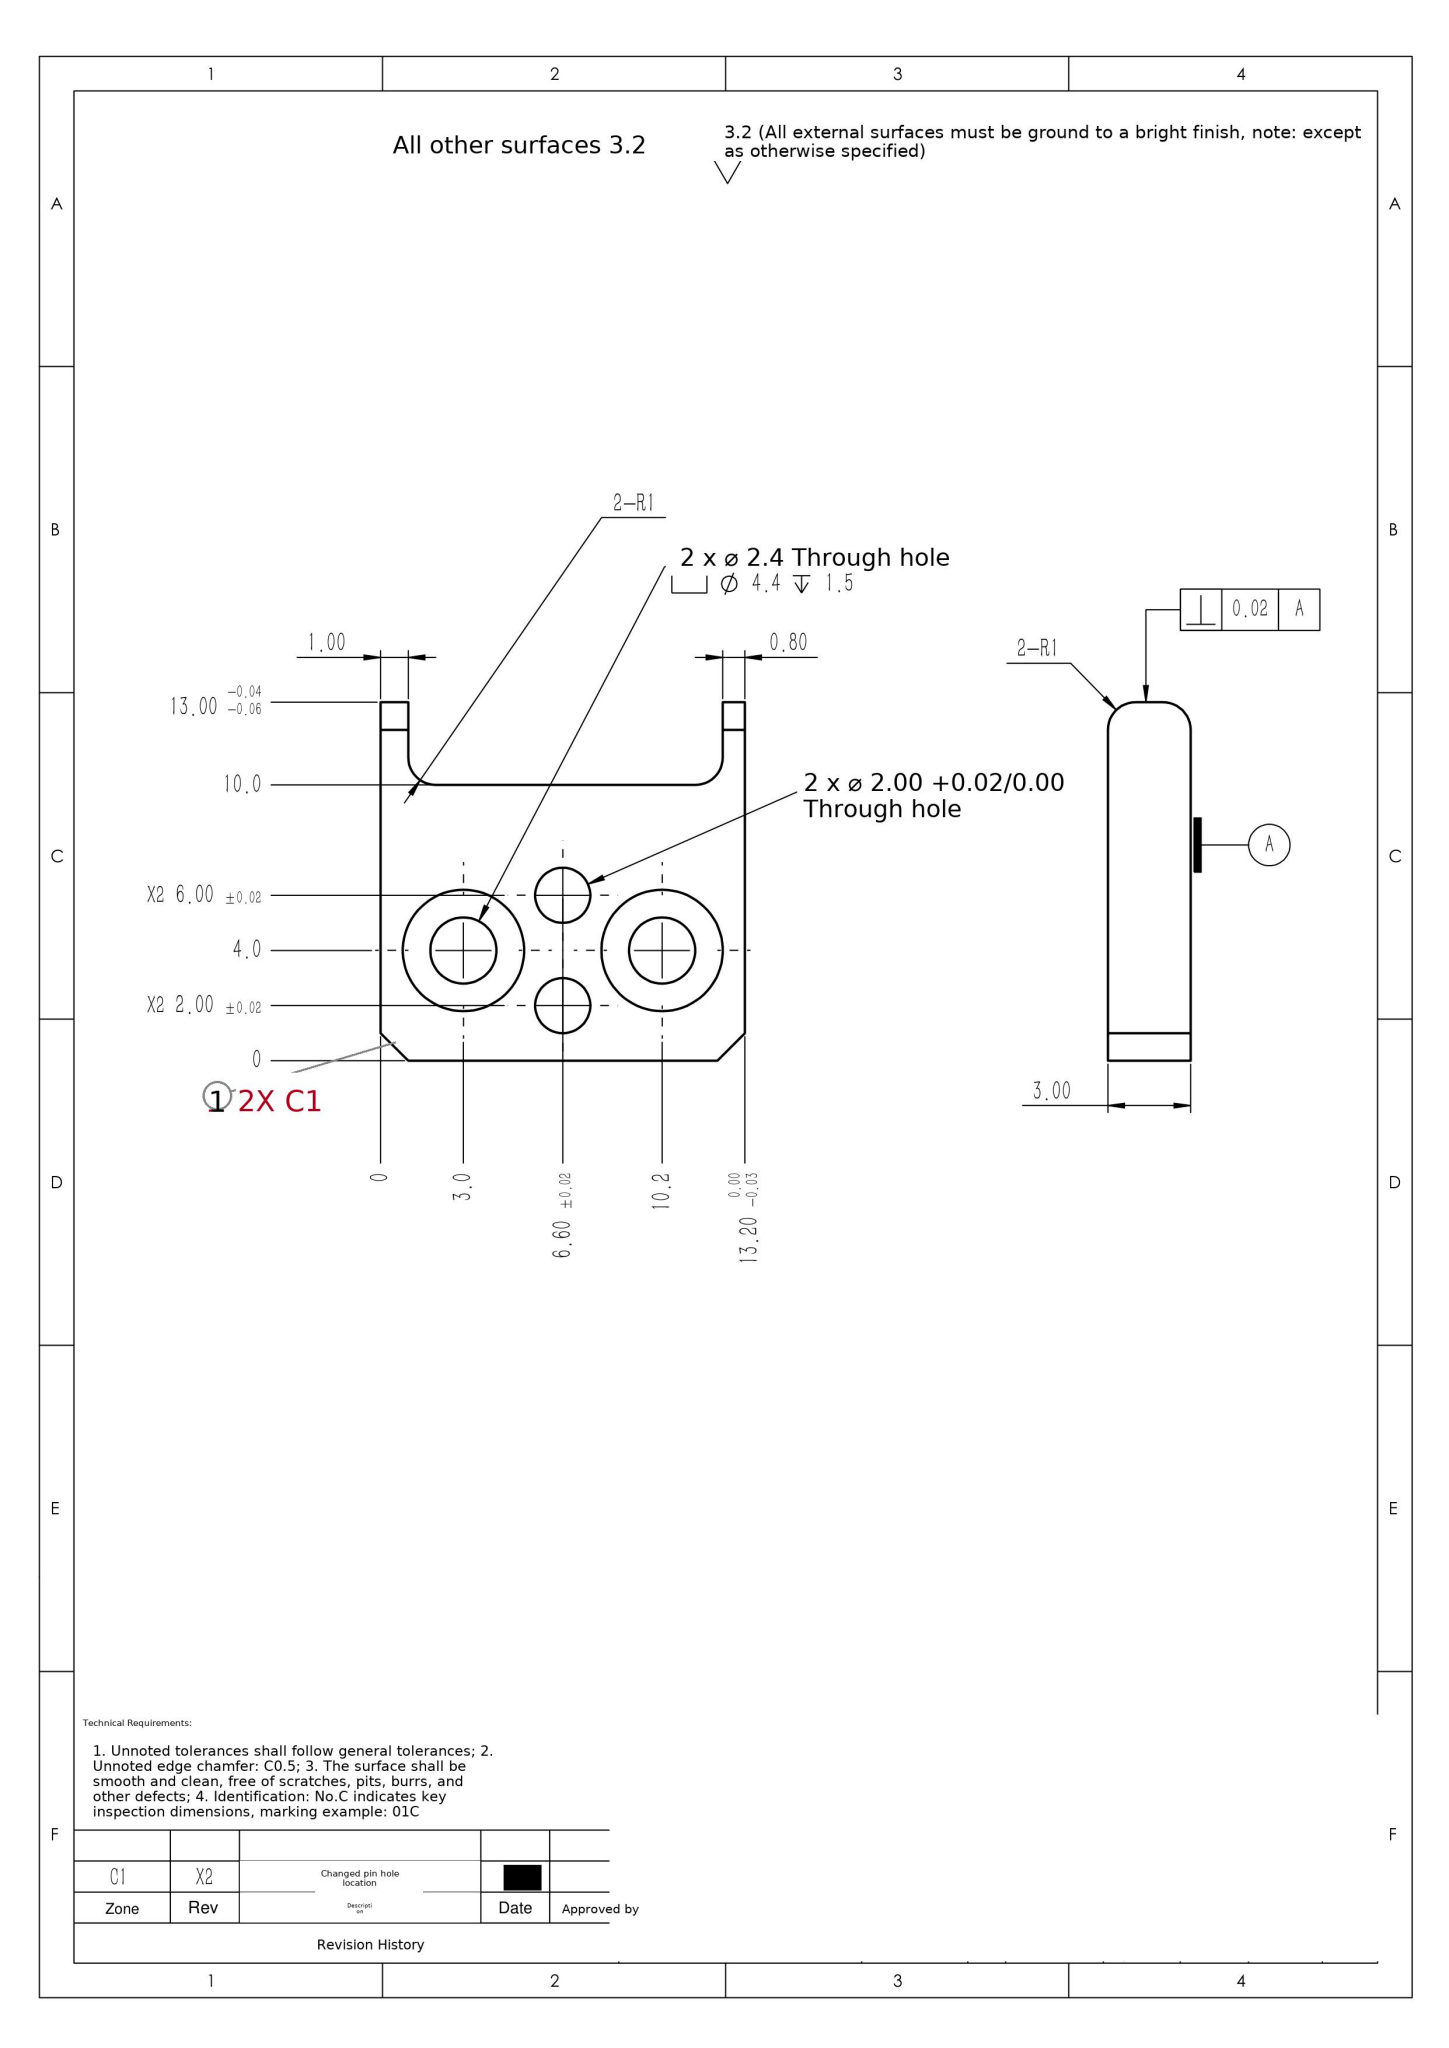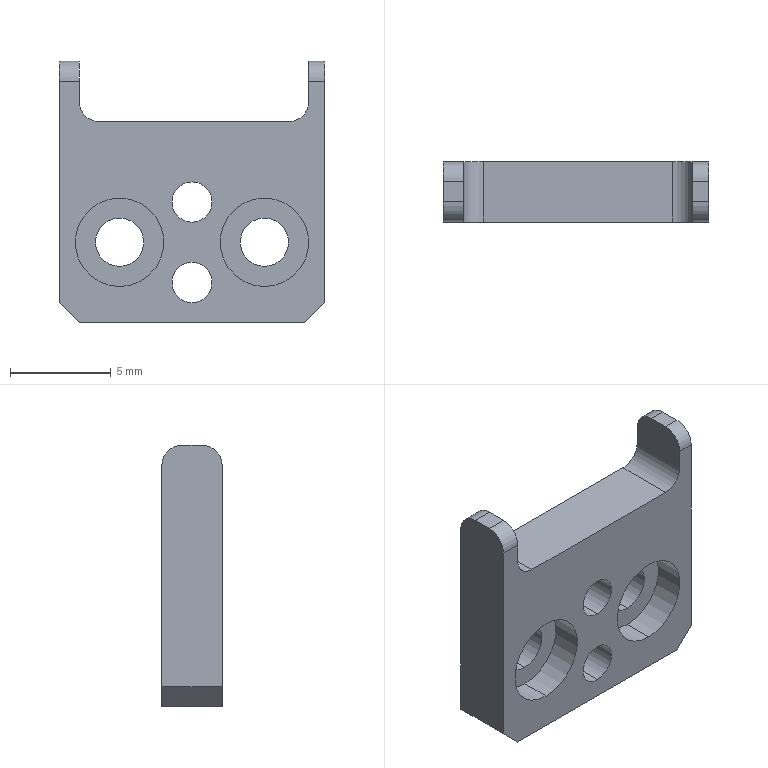Part | SolidWorks | mm | 1 solid | 32 faces | box 13.2 x 3 x 13 mm | volume 332 mm3 | cylinder 18 | plane 14 | commonest cylinder face diameters 2 x10 4.4 x4 2.4 x4
STEP:
#1=CARTESIAN_POINT('',(0.,3.,0.5));
#2=VERTEX_POINT('',#1);
#3=CARTESIAN_POINT('',(0.,3.,-1.5));
#4=VERTEX_POINT('',#3);
#5=CARTESIAN_POINT('',(0.,3.,-0.5));
#6=DIRECTION('',(0.,-1.,0.));
#7=DIRECTION('',(0.,0.,-1.));
#8=AXIS2_PLACEMENT_3D('',#5,#6,#7);
#9=CIRCLE('',#8,1.);
#10=EDGE_CURVE('',#2,#4,#9,.T.);
#11=ORIENTED_EDGE('',*,*,#10,.F.);
#12=CARTESIAN_POINT('',(0.,-0.,0.5));
#13=VERTEX_POINT('',#12);
#14=CARTESIAN_POINT('',(0.,0.,0.5));
#15=DIRECTION('',(0.,-1.,0.));
#16=VECTOR('',#15,1000.);
#17=LINE('',#14,#16);
#18=EDGE_CURVE('',#2,#13,#17,.T.);
#19=ORIENTED_EDGE('',*,*,#18,.T.);
#20=CARTESIAN_POINT('',(0.,-0.,-1.5));
#21=VERTEX_POINT('',#20);
#22=CARTESIAN_POINT('',(0.,-0.,-0.5));
#23=DIRECTION('',(0.,-1.,0.));
#24=DIRECTION('',(0.,0.,-1.));
#25=AXIS2_PLACEMENT_3D('',#22,#23,#24);
#26=CIRCLE('',#25,1.);
#27=EDGE_CURVE('',#13,#21,#26,.T.);
#28=ORIENTED_EDGE('',*,*,#27,.T.);
#29=CARTESIAN_POINT('',(0.,0.,-1.5));
#30=DIRECTION('',(0.,-1.,0.));
#31=VECTOR('',#30,1000.);
#32=LINE('',#29,#31);
#33=EDGE_CURVE('',#4,#21,#32,.T.);
#34=ORIENTED_EDGE('',*,*,#33,.F.);
#35=EDGE_LOOP('',(#11,#19,#28,#34));
#36=FACE_OUTER_BOUND('',#35,.T.);
#37=CARTESIAN_POINT('',(0.,0.,-0.5));
#38=DIRECTION('',(0.,-1.,0.));
#39=DIRECTION('',(0.,0.,-1.));
#40=AXIS2_PLACEMENT_3D('',#37,#38,#39);
#41=CYLINDRICAL_SURFACE('',#40,1.);
#42=ADVANCED_FACE('',(#36),#41,.F.);
#43=CARTESIAN_POINT('',(0.,3.,-3.5));
#44=VERTEX_POINT('',#43);
#45=CARTESIAN_POINT('',(0.,3.,-5.5));
#46=VERTEX_POINT('',#45);
#47=CARTESIAN_POINT('',(0.,3.,-4.5));
#48=DIRECTION('',(0.,-1.,0.));
#49=DIRECTION('',(0.,0.,-1.));
#50=AXIS2_PLACEMENT_3D('',#47,#48,#49);
#51=CIRCLE('',#50,1.);
#52=EDGE_CURVE('',#44,#46,#51,.T.);
#53=ORIENTED_EDGE('',*,*,#52,.F.);
#54=CARTESIAN_POINT('',(0.,-0.,-3.5));
#55=VERTEX_POINT('',#54);
#56=CARTESIAN_POINT('',(0.,0.,-3.5));
#57=DIRECTION('',(0.,-1.,0.));
#58=VECTOR('',#57,1000.);
#59=LINE('',#56,#58);
#60=EDGE_CURVE('',#44,#55,#59,.T.);
#61=ORIENTED_EDGE('',*,*,#60,.T.);
#62=CARTESIAN_POINT('',(0.,-0.,-5.5));
#63=VERTEX_POINT('',#62);
#64=CARTESIAN_POINT('',(0.,-0.,-4.5));
#65=DIRECTION('',(0.,-1.,0.));
#66=DIRECTION('',(0.,0.,-1.));
#67=AXIS2_PLACEMENT_3D('',#64,#65,#66);
#68=CIRCLE('',#67,1.);
#69=EDGE_CURVE('',#55,#63,#68,.T.);
#70=ORIENTED_EDGE('',*,*,#69,.T.);
#71=CARTESIAN_POINT('',(0.,0.,-5.5));
#72=DIRECTION('',(0.,-1.,0.));
#73=VECTOR('',#72,1000.);
#74=LINE('',#71,#73);
#75=EDGE_CURVE('',#46,#63,#74,.T.);
#76=ORIENTED_EDGE('',*,*,#75,.F.);
#77=EDGE_LOOP('',(#53,#61,#70,#76));
#78=FACE_OUTER_BOUND('',#77,.T.);
#79=CARTESIAN_POINT('',(0.,0.,-4.5));
#80=DIRECTION('',(0.,-1.,0.));
#81=DIRECTION('',(0.,0.,-1.));
#82=AXIS2_PLACEMENT_3D('',#79,#80,#81);
#83=CYLINDRICAL_SURFACE('',#82,1.);
#84=ADVANCED_FACE('',(#78),#83,.F.);
#85=CARTESIAN_POINT('',(-3.6,1.5,-0.3));
#86=VERTEX_POINT('',#85);
#87=CARTESIAN_POINT('',(-3.6,1.5,-4.7));
#88=VERTEX_POINT('',#87);
#89=CARTESIAN_POINT('',(-3.6,1.5,-2.5));
#90=DIRECTION('',(0.,-1.,0.));
#91=DIRECTION('',(0.,0.,-1.));
#92=AXIS2_PLACEMENT_3D('',#89,#90,#91);
#93=CIRCLE('',#92,2.2);
#94=EDGE_CURVE('',#86,#88,#93,.T.);
#95=ORIENTED_EDGE('',*,*,#94,.F.);
#96=CARTESIAN_POINT('',(-3.6,0.,-0.3));
#97=VERTEX_POINT('',#96);
#98=CARTESIAN_POINT('',(-3.6,0.,-0.3));
#99=DIRECTION('',(0.,-1.,0.));
#100=VECTOR('',#99,1000.);
#101=LINE('',#98,#100);
#102=EDGE_CURVE('',#86,#97,#101,.T.);
#103=ORIENTED_EDGE('',*,*,#102,.T.);
#104=CARTESIAN_POINT('',(-3.6,0.,-4.7));
#105=VERTEX_POINT('',#104);
#106=CARTESIAN_POINT('',(-3.6,0.,-2.5));
#107=DIRECTION('',(0.,-1.,0.));
#108=DIRECTION('',(0.,0.,-1.));
#109=AXIS2_PLACEMENT_3D('',#106,#107,#108);
#110=CIRCLE('',#109,2.2);
#111=EDGE_CURVE('',#97,#105,#110,.T.);
#112=ORIENTED_EDGE('',*,*,#111,.T.);
#113=CARTESIAN_POINT('',(-3.6,0.,-4.7));
#114=DIRECTION('',(0.,-1.,0.));
#115=VECTOR('',#114,1000.);
#116=LINE('',#113,#115);
#117=EDGE_CURVE('',#88,#105,#116,.T.);
#118=ORIENTED_EDGE('',*,*,#117,.F.);
#119=EDGE_LOOP('',(#95,#103,#112,#118));
#120=FACE_OUTER_BOUND('',#119,.T.);
#121=CARTESIAN_POINT('',(-3.6,0.,-2.5));
#122=DIRECTION('',(0.,-1.,0.));
#123=DIRECTION('',(0.,0.,-1.));
#124=AXIS2_PLACEMENT_3D('',#121,#122,#123);
#125=CYLINDRICAL_SURFACE('',#124,2.2);
#126=ADVANCED_FACE('',(#120),#125,.F.);
#127=CARTESIAN_POINT('',(-3.6,3.,-1.3));
#128=VERTEX_POINT('',#127);
#129=CARTESIAN_POINT('',(-3.6,3.,-3.7));
#130=VERTEX_POINT('',#129);
#131=CARTESIAN_POINT('',(-3.6,3.,-2.5));
#132=DIRECTION('',(0.,-1.,0.));
#133=DIRECTION('',(0.,0.,-1.));
#134=AXIS2_PLACEMENT_3D('',#131,#132,#133);
#135=CIRCLE('',#134,1.2);
#136=EDGE_CURVE('',#128,#130,#135,.T.);
#137=ORIENTED_EDGE('',*,*,#136,.F.);
#138=CARTESIAN_POINT('',(-3.6,1.5,-1.3));
#139=VERTEX_POINT('',#138);
#140=CARTESIAN_POINT('',(-3.6,0.,-1.3));
#141=DIRECTION('',(0.,-1.,0.));
#142=VECTOR('',#141,1000.);
#143=LINE('',#140,#142);
#144=EDGE_CURVE('',#128,#139,#143,.T.);
#145=ORIENTED_EDGE('',*,*,#144,.T.);
#146=CARTESIAN_POINT('',(-3.6,1.5,-3.7));
#147=VERTEX_POINT('',#146);
#148=CARTESIAN_POINT('',(-3.6,1.5,-2.5));
#149=DIRECTION('',(0.,-1.,0.));
#150=DIRECTION('',(0.,0.,-1.));
#151=AXIS2_PLACEMENT_3D('',#148,#149,#150);
#152=CIRCLE('',#151,1.2);
#153=EDGE_CURVE('',#139,#147,#152,.T.);
#154=ORIENTED_EDGE('',*,*,#153,.T.);
#155=CARTESIAN_POINT('',(-3.6,0.,-3.7));
#156=DIRECTION('',(0.,-1.,0.));
#157=VECTOR('',#156,1000.);
#158=LINE('',#155,#157);
#159=EDGE_CURVE('',#130,#147,#158,.T.);
#160=ORIENTED_EDGE('',*,*,#159,.F.);
#161=EDGE_LOOP('',(#137,#145,#154,#160));
#162=FACE_OUTER_BOUND('',#161,.T.);
#163=CARTESIAN_POINT('',(-3.6,0.,-2.5));
#164=DIRECTION('',(0.,-1.,0.));
#165=DIRECTION('',(0.,0.,-1.));
#166=AXIS2_PLACEMENT_3D('',#163,#164,#165);
#167=CYLINDRICAL_SURFACE('',#166,1.2);
#168=ADVANCED_FACE('',(#162),#167,.F.);
#169=CARTESIAN_POINT('',(3.6,1.5,-0.3));
#170=VERTEX_POINT('',#169);
#171=CARTESIAN_POINT('',(3.6,1.5,-4.7));
#172=VERTEX_POINT('',#171);
#173=CARTESIAN_POINT('',(3.6,1.5,-2.5));
#174=DIRECTION('',(0.,-1.,0.));
#175=DIRECTION('',(0.,0.,-1.));
#176=AXIS2_PLACEMENT_3D('',#173,#174,#175);
#177=CIRCLE('',#176,2.2);
#178=EDGE_CURVE('',#170,#172,#177,.T.);
#179=ORIENTED_EDGE('',*,*,#178,.F.);
#180=CARTESIAN_POINT('',(3.6,0.,-0.3));
#181=VERTEX_POINT('',#180);
#182=CARTESIAN_POINT('',(3.6,0.,-0.3));
#183=DIRECTION('',(0.,-1.,0.));
#184=VECTOR('',#183,1000.);
#185=LINE('',#182,#184);
#186=EDGE_CURVE('',#170,#181,#185,.T.);
#187=ORIENTED_EDGE('',*,*,#186,.T.);
#188=CARTESIAN_POINT('',(3.6,0.,-4.7));
#189=VERTEX_POINT('',#188);
#190=CARTESIAN_POINT('',(3.6,0.,-2.5));
#191=DIRECTION('',(0.,-1.,0.));
#192=DIRECTION('',(0.,0.,-1.));
#193=AXIS2_PLACEMENT_3D('',#190,#191,#192);
#194=CIRCLE('',#193,2.2);
#195=EDGE_CURVE('',#181,#189,#194,.T.);
#196=ORIENTED_EDGE('',*,*,#195,.T.);
#197=CARTESIAN_POINT('',(3.6,0.,-4.7));
#198=DIRECTION('',(0.,-1.,0.));
#199=VECTOR('',#198,1000.);
#200=LINE('',#197,#199);
#201=EDGE_CURVE('',#172,#189,#200,.T.);
#202=ORIENTED_EDGE('',*,*,#201,.F.);
#203=EDGE_LOOP('',(#179,#187,#196,#202));
#204=FACE_OUTER_BOUND('',#203,.T.);
#205=CARTESIAN_POINT('',(3.6,0.,-2.5));
#206=DIRECTION('',(0.,-1.,0.));
#207=DIRECTION('',(0.,0.,-1.));
#208=AXIS2_PLACEMENT_3D('',#205,#206,#207);
#209=CYLINDRICAL_SURFACE('',#208,2.2);
#210=ADVANCED_FACE('',(#204),#209,.F.);
#211=CARTESIAN_POINT('',(3.6,3.,-1.3));
#212=VERTEX_POINT('',#211);
#213=CARTESIAN_POINT('',(3.6,3.,-3.7));
#214=VERTEX_POINT('',#213);
#215=CARTESIAN_POINT('',(3.6,3.,-2.5));
#216=DIRECTION('',(0.,-1.,0.));
#217=DIRECTION('',(0.,0.,-1.));
#218=AXIS2_PLACEMENT_3D('',#215,#216,#217);
#219=CIRCLE('',#218,1.2);
#220=EDGE_CURVE('',#212,#214,#219,.T.);
#221=ORIENTED_EDGE('',*,*,#220,.F.);
#222=CARTESIAN_POINT('',(3.6,1.5,-1.3));
#223=VERTEX_POINT('',#222);
#224=CARTESIAN_POINT('',(3.6,0.,-1.3));
#225=DIRECTION('',(0.,-1.,0.));
#226=VECTOR('',#225,1000.);
#227=LINE('',#224,#226);
#228=EDGE_CURVE('',#212,#223,#227,.T.);
#229=ORIENTED_EDGE('',*,*,#228,.T.);
#230=CARTESIAN_POINT('',(3.6,1.5,-3.7));
#231=VERTEX_POINT('',#230);
#232=CARTESIAN_POINT('',(3.6,1.5,-2.5));
#233=DIRECTION('',(0.,-1.,0.));
#234=DIRECTION('',(0.,0.,-1.));
#235=AXIS2_PLACEMENT_3D('',#232,#233,#234);
#236=CIRCLE('',#235,1.2);
#237=EDGE_CURVE('',#223,#231,#236,.T.);
#238=ORIENTED_EDGE('',*,*,#237,.T.);
#239=CARTESIAN_POINT('',(3.6,0.,-3.7));
#240=DIRECTION('',(0.,-1.,0.));
#241=VECTOR('',#240,1000.);
#242=LINE('',#239,#241);
#243=EDGE_CURVE('',#214,#231,#242,.T.);
#244=ORIENTED_EDGE('',*,*,#243,.F.);
#245=EDGE_LOOP('',(#221,#229,#238,#244));
#246=FACE_OUTER_BOUND('',#245,.T.);
#247=CARTESIAN_POINT('',(3.6,0.,-2.5));
#248=DIRECTION('',(0.,-1.,0.));
#249=DIRECTION('',(0.,0.,-1.));
#250=AXIS2_PLACEMENT_3D('',#247,#248,#249);
#251=CYLINDRICAL_SURFACE('',#250,1.2);
#252=ADVANCED_FACE('',(#246),#251,.F.);
#253=CARTESIAN_POINT('',(0.,3.,-0.5));
#254=DIRECTION('',(0.,-1.,0.));
#255=DIRECTION('',(0.,0.,-1.));
#256=AXIS2_PLACEMENT_3D('',#253,#254,#255);
#257=CIRCLE('',#256,1.);
#258=EDGE_CURVE('',#4,#2,#257,.T.);
#259=ORIENTED_EDGE('',*,*,#258,.T.);
#260=ORIENTED_EDGE('',*,*,#10,.T.);
#261=EDGE_LOOP('',(#259,#260));
#262=FACE_BOUND('',#261,.T.);
#263=CARTESIAN_POINT('',(0.,3.,-4.5));
#264=DIRECTION('',(0.,-1.,0.));
#265=DIRECTION('',(0.,0.,-1.));
#266=AXIS2_PLACEMENT_3D('',#263,#264,#265);
#267=CIRCLE('',#266,1.);
#268=EDGE_CURVE('',#46,#44,#267,.T.);
#269=ORIENTED_EDGE('',*,*,#268,.T.);
#270=ORIENTED_EDGE('',*,*,#52,.T.);
#271=EDGE_LOOP('',(#269,#270));
#272=FACE_BOUND('',#271,.T.);
#273=CARTESIAN_POINT('',(6.6,3.,5.5));
#274=VERTEX_POINT('',#273);
#275=CARTESIAN_POINT('',(6.6,3.,-5.5));
#276=VERTEX_POINT('',#275);
#277=CARTESIAN_POINT('',(6.6,3.,-6.5));
#278=DIRECTION('',(-0.,0.,-1.));
#279=VECTOR('',#278,1000.);
#280=LINE('',#277,#279);
#281=EDGE_CURVE('',#274,#276,#280,.T.);
#282=ORIENTED_EDGE('',*,*,#281,.T.);
#283=CARTESIAN_POINT('',(5.6,3.,-6.5));
#284=VERTEX_POINT('',#283);
#285=CARTESIAN_POINT('',(6.05,3.,-6.05));
#286=DIRECTION('',(-0.7071,0.,-0.7071));
#287=VECTOR('',#286,1000.);
#288=LINE('',#285,#287);
#289=EDGE_CURVE('',#276,#284,#288,.T.);
#290=ORIENTED_EDGE('',*,*,#289,.T.);
#291=CARTESIAN_POINT('',(-5.6,3.,-6.5));
#292=VERTEX_POINT('',#291);
#293=CARTESIAN_POINT('',(-6.6,3.,-6.5));
#294=DIRECTION('',(-1.,0.,0.));
#295=VECTOR('',#294,1000.);
#296=LINE('',#293,#295);
#297=EDGE_CURVE('',#284,#292,#296,.T.);
#298=ORIENTED_EDGE('',*,*,#297,.T.);
#299=CARTESIAN_POINT('',(-6.6,3.,-5.5));
#300=VERTEX_POINT('',#299);
#301=CARTESIAN_POINT('',(-6.05,3.,-6.05));
#302=DIRECTION('',(-0.7071,0.,0.7071));
#303=VECTOR('',#302,1000.);
#304=LINE('',#301,#303);
#305=EDGE_CURVE('',#292,#300,#304,.T.);
#306=ORIENTED_EDGE('',*,*,#305,.T.);
#307=CARTESIAN_POINT('',(-6.6,3.,5.5));
#308=VERTEX_POINT('',#307);
#309=CARTESIAN_POINT('',(-6.6,3.,-6.5));
#310=DIRECTION('',(0.,0.,1.));
#311=VECTOR('',#310,1000.);
#312=LINE('',#309,#311);
#313=EDGE_CURVE('',#300,#308,#312,.T.);
#314=ORIENTED_EDGE('',*,*,#313,.T.);
#315=CARTESIAN_POINT('',(-5.6,3.,5.5));
#316=VERTEX_POINT('',#315);
#317=CARTESIAN_POINT('',(-5.6,3.,5.5));
#318=DIRECTION('',(1.,0.,0.));
#319=VECTOR('',#318,1000.);
#320=LINE('',#317,#319);
#321=EDGE_CURVE('',#308,#316,#320,.T.);
#322=ORIENTED_EDGE('',*,*,#321,.T.);
#323=CARTESIAN_POINT('',(-5.6,3.,4.5));
#324=VERTEX_POINT('',#323);
#325=CARTESIAN_POINT('',(-5.6,3.,6.5));
#326=DIRECTION('',(0.,0.,-1.));
#327=VECTOR('',#326,1000.);
#328=LINE('',#325,#327);
#329=EDGE_CURVE('',#316,#324,#328,.T.);
#330=ORIENTED_EDGE('',*,*,#329,.T.);
#331=CARTESIAN_POINT('',(-4.6,3.,3.5));
#332=VERTEX_POINT('',#331);
#333=CARTESIAN_POINT('',(-4.6,3.,4.5));
#334=DIRECTION('',(0.,-1.,0.));
#335=DIRECTION('',(0.,0.,1.));
#336=AXIS2_PLACEMENT_3D('',#333,#334,#335);
#337=CIRCLE('',#336,1.);
#338=EDGE_CURVE('',#324,#332,#337,.T.);
#339=ORIENTED_EDGE('',*,*,#338,.T.);
#340=CARTESIAN_POINT('',(4.8,3.,3.5));
#341=VERTEX_POINT('',#340);
#342=CARTESIAN_POINT('',(5.8,3.,3.5));
#343=DIRECTION('',(1.,0.,0.));
#344=VECTOR('',#343,1000.);
#345=LINE('',#342,#344);
#346=EDGE_CURVE('',#332,#341,#345,.T.);
#347=ORIENTED_EDGE('',*,*,#346,.T.);
#348=CARTESIAN_POINT('',(5.8,3.,4.5));
#349=VERTEX_POINT('',#348);
#350=CARTESIAN_POINT('',(4.8,3.,4.5));
#351=DIRECTION('',(0.,-1.,0.));
#352=DIRECTION('',(0.,0.,1.));
#353=AXIS2_PLACEMENT_3D('',#350,#351,#352);
#354=CIRCLE('',#353,1.);
#355=EDGE_CURVE('',#341,#349,#354,.T.);
#356=ORIENTED_EDGE('',*,*,#355,.T.);
#357=CARTESIAN_POINT('',(5.8,3.,5.5));
#358=VERTEX_POINT('',#357);
#359=CARTESIAN_POINT('',(5.8,3.,6.5));
#360=DIRECTION('',(0.,0.,1.));
#361=VECTOR('',#360,1000.);
#362=LINE('',#359,#361);
#363=EDGE_CURVE('',#349,#358,#362,.T.);
#364=ORIENTED_EDGE('',*,*,#363,.T.);
#365=CARTESIAN_POINT('',(6.6,3.,5.5));
#366=DIRECTION('',(1.,0.,0.));
#367=VECTOR('',#366,1000.);
#368=LINE('',#365,#367);
#369=EDGE_CURVE('',#358,#274,#368,.T.);
#370=ORIENTED_EDGE('',*,*,#369,.T.);
#371=EDGE_LOOP('',(#282,#290,#298,#306,#314,#322,#330,#339,#347,#356,#364,#370));
#372=FACE_OUTER_BOUND('',#371,.T.);
#373=CARTESIAN_POINT('',(3.6,3.,-2.5));
#374=DIRECTION('',(0.,-1.,0.));
#375=DIRECTION('',(0.,0.,-1.));
#376=AXIS2_PLACEMENT_3D('',#373,#374,#375);
#377=CIRCLE('',#376,1.2);
#378=EDGE_CURVE('',#214,#212,#377,.T.);
#379=ORIENTED_EDGE('',*,*,#378,.T.);
#380=ORIENTED_EDGE('',*,*,#220,.T.);
#381=EDGE_LOOP('',(#379,#380));
#382=FACE_BOUND('',#381,.T.);
#383=CARTESIAN_POINT('',(-3.6,3.,-2.5));
#384=DIRECTION('',(0.,-1.,0.));
#385=DIRECTION('',(0.,0.,-1.));
#386=AXIS2_PLACEMENT_3D('',#383,#384,#385);
#387=CIRCLE('',#386,1.2);
#388=EDGE_CURVE('',#130,#128,#387,.T.);
#389=ORIENTED_EDGE('',*,*,#388,.T.);
#390=ORIENTED_EDGE('',*,*,#136,.T.);
#391=EDGE_LOOP('',(#389,#390));
#392=FACE_BOUND('',#391,.T.);
#393=CARTESIAN_POINT('',(0.,3.,0.));
#394=DIRECTION('',(0.,1.,0.));
#395=DIRECTION('',(0.,0.,1.));
#396=AXIS2_PLACEMENT_3D('',#393,#394,#395);
#397=PLANE('',#396);
#398=ADVANCED_FACE('',(#262,#272,#372,#382,#392),#397,.T.);
#399=CARTESIAN_POINT('',(6.6,2.,6.5));
#400=VERTEX_POINT('',#399);
#401=CARTESIAN_POINT('',(6.6,1.,6.5));
#402=VERTEX_POINT('',#401);
#403=CARTESIAN_POINT('',(6.6,3.,6.5));
#404=DIRECTION('',(0.,-1.,0.));
#405=VECTOR('',#404,1000.);
#406=LINE('',#403,#405);
#407=EDGE_CURVE('',#400,#402,#406,.T.);
#408=ORIENTED_EDGE('',*,*,#407,.F.);
#409=CARTESIAN_POINT('',(5.8,2.,6.5));
#410=VERTEX_POINT('',#409);
#411=CARTESIAN_POINT('',(5.8,2.,6.5));
#412=DIRECTION('',(-1.,0.,0.));
#413=VECTOR('',#412,1000.);
#414=LINE('',#411,#413);
#415=EDGE_CURVE('',#400,#410,#414,.T.);
#416=ORIENTED_EDGE('',*,*,#415,.T.);
#417=CARTESIAN_POINT('',(5.8,1.,6.5));
#418=VERTEX_POINT('',#417);
#419=CARTESIAN_POINT('',(5.8,3.,6.5));
#420=DIRECTION('',(0.,-1.,0.));
#421=VECTOR('',#420,1000.);
#422=LINE('',#419,#421);
#423=EDGE_CURVE('',#410,#418,#422,.T.);
#424=ORIENTED_EDGE('',*,*,#423,.T.);
#425=CARTESIAN_POINT('',(-6.6,1.,6.5));
#426=DIRECTION('',(1.,0.,0.));
#427=VECTOR('',#426,1000.);
#428=LINE('',#425,#427);
#429=EDGE_CURVE('',#418,#402,#428,.T.);
#430=ORIENTED_EDGE('',*,*,#429,.T.);
#431=EDGE_LOOP('',(#408,#416,#424,#430));
#432=FACE_OUTER_BOUND('',#431,.T.);
#433=CARTESIAN_POINT('',(-6.6,3.,6.5));
#434=DIRECTION('',(0.,0.,-1.));
#435=DIRECTION('',(-1.,0.,0.));
#436=AXIS2_PLACEMENT_3D('',#433,#434,#435);
#437=PLANE('',#436);
#438=ADVANCED_FACE('',(#432),#437,.F.);
#439=CARTESIAN_POINT('',(6.6,0.,5.5));
#440=VERTEX_POINT('',#439);
#441=CARTESIAN_POINT('',(6.6,0.,-5.5));
#442=VERTEX_POINT('',#441);
#443=CARTESIAN_POINT('',(6.6,0.,-6.5));
#444=DIRECTION('',(-0.,0.,-1.));
#445=VECTOR('',#444,1000.);
#446=LINE('',#443,#445);
#447=EDGE_CURVE('',#440,#442,#446,.T.);
#448=ORIENTED_EDGE('',*,*,#447,.T.);
#449=CARTESIAN_POINT('',(6.6,3.,-5.5));
#450=DIRECTION('',(0.,1.,0.));
#451=VECTOR('',#450,1000.);
#452=LINE('',#449,#451);
#453=EDGE_CURVE('',#442,#276,#452,.T.);
#454=ORIENTED_EDGE('',*,*,#453,.T.);
#455=ORIENTED_EDGE('',*,*,#281,.F.);
#456=CARTESIAN_POINT('',(6.6,2.,5.5));
#457=DIRECTION('',(1.,0.,-0.));
#458=DIRECTION('',(0.,0.,1.));
#459=AXIS2_PLACEMENT_3D('',#456,#457,#458);
#460=CIRCLE('',#459,1.);
#461=EDGE_CURVE('',#274,#400,#460,.T.);
#462=ORIENTED_EDGE('',*,*,#461,.T.);
#463=ORIENTED_EDGE('',*,*,#407,.T.);
#464=CARTESIAN_POINT('',(6.6,1.,5.5));
#465=DIRECTION('',(1.,0.,-0.));
#466=DIRECTION('',(0.,0.,1.));
#467=AXIS2_PLACEMENT_3D('',#464,#465,#466);
#468=CIRCLE('',#467,1.);
#469=EDGE_CURVE('',#402,#440,#468,.T.);
#470=ORIENTED_EDGE('',*,*,#469,.T.);
#471=EDGE_LOOP('',(#448,#454,#455,#462,#463,#470));
#472=FACE_OUTER_BOUND('',#471,.T.);
#473=CARTESIAN_POINT('',(6.6,3.,-6.5));
#474=DIRECTION('',(-1.,0.,0.));
#475=DIRECTION('',(0.,0.,1.));
#476=AXIS2_PLACEMENT_3D('',#473,#474,#475);
#477=PLANE('',#476);
#478=ADVANCED_FACE('',(#472),#477,.F.);
#479=ORIENTED_EDGE('',*,*,#297,.F.);
#480=CARTESIAN_POINT('',(5.6,0.,-6.5));
#481=VERTEX_POINT('',#480);
#482=CARTESIAN_POINT('',(5.6,3.,-6.5));
#483=DIRECTION('',(0.,-1.,0.));
#484=VECTOR('',#483,1000.);
#485=LINE('',#482,#484);
#486=EDGE_CURVE('',#284,#481,#485,.T.);
#487=ORIENTED_EDGE('',*,*,#486,.T.);
#488=CARTESIAN_POINT('',(-5.6,0.,-6.5));
#489=VERTEX_POINT('',#488);
#490=CARTESIAN_POINT('',(-6.6,0.,-6.5));
#491=DIRECTION('',(-1.,0.,0.));
#492=VECTOR('',#491,1000.);
#493=LINE('',#490,#492);
#494=EDGE_CURVE('',#481,#489,#493,.T.);
#495=ORIENTED_EDGE('',*,*,#494,.T.);
#496=CARTESIAN_POINT('',(-5.6,3.,-6.5));
#497=DIRECTION('',(0.,1.,0.));
#498=VECTOR('',#497,1000.);
#499=LINE('',#496,#498);
#500=EDGE_CURVE('',#489,#292,#499,.T.);
#501=ORIENTED_EDGE('',*,*,#500,.T.);
#502=EDGE_LOOP('',(#479,#487,#495,#501));
#503=FACE_OUTER_BOUND('',#502,.T.);
#504=CARTESIAN_POINT('',(-6.6,3.,-6.5));
#505=DIRECTION('',(0.,0.,1.));
#506=DIRECTION('',(1.,0.,0.));
#507=AXIS2_PLACEMENT_3D('',#504,#505,#506);
#508=PLANE('',#507);
#509=ADVANCED_FACE('',(#503),#508,.F.);
#510=ORIENTED_EDGE('',*,*,#313,.F.);
#511=CARTESIAN_POINT('',(-6.6,0.,-5.5));
#512=VERTEX_POINT('',#511);
#513=CARTESIAN_POINT('',(-6.6,3.,-5.5));
#514=DIRECTION('',(0.,-1.,0.));
#515=VECTOR('',#514,1000.);
#516=LINE('',#513,#515);
#517=EDGE_CURVE('',#300,#512,#516,.T.);
#518=ORIENTED_EDGE('',*,*,#517,.T.);
#519=CARTESIAN_POINT('',(-6.6,0.,5.5));
#520=VERTEX_POINT('',#519);
#521=CARTESIAN_POINT('',(-6.6,0.,-6.5));
#522=DIRECTION('',(0.,0.,1.));
#523=VECTOR('',#522,1000.);
#524=LINE('',#521,#523);
#525=EDGE_CURVE('',#512,#520,#524,.T.);
#526=ORIENTED_EDGE('',*,*,#525,.T.);
#527=CARTESIAN_POINT('',(-6.6,1.,6.5));
#528=VERTEX_POINT('',#527);
#529=CARTESIAN_POINT('',(-6.6,1.,5.5));
#530=DIRECTION('',(-1.,0.,0.));
#531=DIRECTION('',(0.,0.,-1.));
#532=AXIS2_PLACEMENT_3D('',#529,#530,#531);
#533=CIRCLE('',#532,1.);
#534=EDGE_CURVE('',#520,#528,#533,.T.);
#535=ORIENTED_EDGE('',*,*,#534,.T.);
#536=CARTESIAN_POINT('',(-6.6,2.,6.5));
#537=VERTEX_POINT('',#536);
#538=CARTESIAN_POINT('',(-6.6,3.,6.5));
#539=DIRECTION('',(0.,-1.,0.));
#540=VECTOR('',#539,1000.);
#541=LINE('',#538,#540);
#542=EDGE_CURVE('',#537,#528,#541,.T.);
#543=ORIENTED_EDGE('',*,*,#542,.F.);
#544=CARTESIAN_POINT('',(-6.6,2.,5.5));
#545=DIRECTION('',(-1.,0.,0.));
#546=DIRECTION('',(0.,0.,-1.));
#547=AXIS2_PLACEMENT_3D('',#544,#545,#546);
#548=CIRCLE('',#547,1.);
#549=EDGE_CURVE('',#537,#308,#548,.T.);
#550=ORIENTED_EDGE('',*,*,#549,.T.);
#551=EDGE_LOOP('',(#510,#518,#526,#535,#543,#550));
#552=FACE_OUTER_BOUND('',#551,.T.);
#553=CARTESIAN_POINT('',(-6.6,3.,-6.5));
#554=DIRECTION('',(1.,0.,-0.));
#555=DIRECTION('',(-0.,0.,-1.));
#556=AXIS2_PLACEMENT_3D('',#553,#554,#555);
#557=PLANE('',#556);
#558=ADVANCED_FACE('',(#552),#557,.F.);
#559=CARTESIAN_POINT('',(-5.6,2.,6.5));
#560=VERTEX_POINT('',#559);
#561=CARTESIAN_POINT('',(-5.6,1.,6.5));
#562=VERTEX_POINT('',#561);
#563=CARTESIAN_POINT('',(-5.6,3.,6.5));
#564=DIRECTION('',(0.,-1.,0.));
#565=VECTOR('',#564,1000.);
#566=LINE('',#563,#565);
#567=EDGE_CURVE('',#560,#562,#566,.T.);
#568=ORIENTED_EDGE('',*,*,#567,.F.);
#569=CARTESIAN_POINT('',(-6.6,2.,6.5));
#570=DIRECTION('',(-1.,0.,0.));
#571=VECTOR('',#570,1000.);
#572=LINE('',#569,#571);
#573=EDGE_CURVE('',#560,#537,#572,.T.);
#574=ORIENTED_EDGE('',*,*,#573,.T.);
#575=ORIENTED_EDGE('',*,*,#542,.T.);
#576=CARTESIAN_POINT('',(-6.6,1.,6.5));
#577=DIRECTION('',(1.,0.,0.));
#578=VECTOR('',#577,1000.);
#579=LINE('',#576,#578);
#580=EDGE_CURVE('',#528,#562,#579,.T.);
#581=ORIENTED_EDGE('',*,*,#580,.T.);
#582=EDGE_LOOP('',(#568,#574,#575,#581));
#583=FACE_OUTER_BOUND('',#582,.T.);
#584=CARTESIAN_POINT('',(-6.6,3.,6.5));
#585=DIRECTION('',(0.,0.,-1.));
#586=DIRECTION('',(-1.,0.,0.));
#587=AXIS2_PLACEMENT_3D('',#584,#585,#586);
#588=PLANE('',#587);
#589=ADVANCED_FACE('',(#583),#588,.F.);
#590=CARTESIAN_POINT('',(0.,-0.,-0.5));
#591=DIRECTION('',(0.,-1.,0.));
#592=DIRECTION('',(0.,0.,-1.));
#593=AXIS2_PLACEMENT_3D('',#590,#591,#592);
#594=CIRCLE('',#593,1.);
#595=EDGE_CURVE('',#21,#13,#594,.T.);
#596=ORIENTED_EDGE('',*,*,#595,.F.);
#597=ORIENTED_EDGE('',*,*,#27,.F.);
#598=EDGE_LOOP('',(#596,#597));
#599=FACE_BOUND('',#598,.T.);
#600=CARTESIAN_POINT('',(0.,-0.,-4.5));
#601=DIRECTION('',(0.,-1.,0.));
#602=DIRECTION('',(0.,0.,-1.));
#603=AXIS2_PLACEMENT_3D('',#600,#601,#602);
#604=CIRCLE('',#603,1.);
#605=EDGE_CURVE('',#63,#55,#604,.T.);
#606=ORIENTED_EDGE('',*,*,#605,.F.);
#607=ORIENTED_EDGE('',*,*,#69,.F.);
#608=EDGE_LOOP('',(#606,#607));
#609=FACE_BOUND('',#608,.T.);
#610=CARTESIAN_POINT('',(-3.6,0.,-2.5));
#611=DIRECTION('',(0.,-1.,0.));
#612=DIRECTION('',(0.,0.,-1.));
#613=AXIS2_PLACEMENT_3D('',#610,#611,#612);
#614=CIRCLE('',#613,2.2);
#615=EDGE_CURVE('',#105,#97,#614,.T.);
#616=ORIENTED_EDGE('',*,*,#615,.F.);
#617=ORIENTED_EDGE('',*,*,#111,.F.);
#618=EDGE_LOOP('',(#616,#617));
#619=FACE_BOUND('',#618,.T.);
#620=CARTESIAN_POINT('',(3.6,0.,-2.5));
#621=DIRECTION('',(0.,-1.,0.));
#622=DIRECTION('',(0.,0.,-1.));
#623=AXIS2_PLACEMENT_3D('',#620,#621,#622);
#624=CIRCLE('',#623,2.2);
#625=EDGE_CURVE('',#189,#181,#624,.T.);
#626=ORIENTED_EDGE('',*,*,#625,.F.);
#627=ORIENTED_EDGE('',*,*,#195,.F.);
#628=EDGE_LOOP('',(#626,#627));
#629=FACE_BOUND('',#628,.T.);
#630=ORIENTED_EDGE('',*,*,#494,.F.);
#631=CARTESIAN_POINT('',(5.6,0.,-6.5));
#632=DIRECTION('',(0.7071,0.,0.7071));
#633=VECTOR('',#632,1000.);
#634=LINE('',#631,#633);
#635=EDGE_CURVE('',#481,#442,#634,.T.);
#636=ORIENTED_EDGE('',*,*,#635,.T.);
#637=ORIENTED_EDGE('',*,*,#447,.F.);
#638=CARTESIAN_POINT('',(5.8,0.,5.5));
#639=VERTEX_POINT('',#638);
#640=CARTESIAN_POINT('',(0.,0.,5.5));
#641=DIRECTION('',(-1.,0.,0.));
#642=VECTOR('',#641,1000.);
#643=LINE('',#640,#642);
#644=EDGE_CURVE('',#440,#639,#643,.T.);
#645=ORIENTED_EDGE('',*,*,#644,.T.);
#646=CARTESIAN_POINT('',(5.8,0.,4.5));
#647=VERTEX_POINT('',#646);
#648=CARTESIAN_POINT('',(5.8,0.,6.5));
#649=DIRECTION('',(0.,0.,1.));
#650=VECTOR('',#649,1000.);
#651=LINE('',#648,#650);
#652=EDGE_CURVE('',#647,#639,#651,.T.);
#653=ORIENTED_EDGE('',*,*,#652,.F.);
#654=CARTESIAN_POINT('',(4.8,0.,3.5));
#655=VERTEX_POINT('',#654);
#656=CARTESIAN_POINT('',(4.8,0.,4.5));
#657=DIRECTION('',(0.,1.,0.));
#658=DIRECTION('',(0.,0.,1.));
#659=AXIS2_PLACEMENT_3D('',#656,#657,#658);
#660=CIRCLE('',#659,1.);
#661=EDGE_CURVE('',#647,#655,#660,.T.);
#662=ORIENTED_EDGE('',*,*,#661,.T.);
#663=CARTESIAN_POINT('',(-4.6,0.,3.5));
#664=VERTEX_POINT('',#663);
#665=CARTESIAN_POINT('',(5.8,0.,3.5));
#666=DIRECTION('',(1.,0.,0.));
#667=VECTOR('',#666,1000.);
#668=LINE('',#665,#667);
#669=EDGE_CURVE('',#664,#655,#668,.T.);
#670=ORIENTED_EDGE('',*,*,#669,.F.);
#671=CARTESIAN_POINT('',(-5.6,0.,4.5));
#672=VERTEX_POINT('',#671);
#673=CARTESIAN_POINT('',(-4.6,0.,4.5));
#674=DIRECTION('',(0.,1.,0.));
#675=DIRECTION('',(0.,0.,1.));
#676=AXIS2_PLACEMENT_3D('',#673,#674,#675);
#677=CIRCLE('',#676,1.);
#678=EDGE_CURVE('',#664,#672,#677,.T.);
#679=ORIENTED_EDGE('',*,*,#678,.T.);
#680=CARTESIAN_POINT('',(-5.6,0.,5.5));
#681=VERTEX_POINT('',#680);
#682=CARTESIAN_POINT('',(-5.6,0.,6.5));
#683=DIRECTION('',(0.,0.,-1.));
#684=VECTOR('',#683,1000.);
#685=LINE('',#682,#684);
#686=EDGE_CURVE('',#681,#672,#685,.T.);
#687=ORIENTED_EDGE('',*,*,#686,.F.);
#688=CARTESIAN_POINT('',(0.,0.,5.5));
#689=DIRECTION('',(-1.,0.,0.));
#690=VECTOR('',#689,1000.);
#691=LINE('',#688,#690);
#692=EDGE_CURVE('',#681,#520,#691,.T.);
#693=ORIENTED_EDGE('',*,*,#692,.T.);
#694=ORIENTED_EDGE('',*,*,#525,.F.);
#695=CARTESIAN_POINT('',(-6.6,0.,-5.5));
#696=DIRECTION('',(0.7071,0.,-0.7071));
#697=VECTOR('',#696,1000.);
#698=LINE('',#695,#697);
#699=EDGE_CURVE('',#512,#489,#698,.T.);
#700=ORIENTED_EDGE('',*,*,#699,.T.);
#701=EDGE_LOOP('',(#630,#636,#637,#645,#653,#662,#670,#679,#687,#693,#694,#700));
#702=FACE_OUTER_BOUND('',#701,.T.);
#703=CARTESIAN_POINT('',(0.,0.,0.));
#704=DIRECTION('',(0.,1.,0.));
#705=DIRECTION('',(0.,0.,1.));
#706=AXIS2_PLACEMENT_3D('',#703,#704,#705);
#707=PLANE('',#706);
#708=ADVANCED_FACE('',(#599,#609,#619,#629,#702),#707,.F.);
#709=ORIENTED_EDGE('',*,*,#423,.F.);
#710=CARTESIAN_POINT('',(5.8,2.,5.5));
#711=DIRECTION('',(-1.,0.,0.));
#712=DIRECTION('',(0.,0.,-1.));
#713=AXIS2_PLACEMENT_3D('',#710,#711,#712);
#714=CIRCLE('',#713,1.);
#715=EDGE_CURVE('',#410,#358,#714,.T.);
#716=ORIENTED_EDGE('',*,*,#715,.T.);
#717=ORIENTED_EDGE('',*,*,#363,.F.);
#718=CARTESIAN_POINT('',(5.8,0.,4.5));
#719=DIRECTION('',(0.,-1.,0.));
#720=VECTOR('',#719,1000.);
#721=LINE('',#718,#720);
#722=EDGE_CURVE('',#349,#647,#721,.T.);
#723=ORIENTED_EDGE('',*,*,#722,.T.);
#724=ORIENTED_EDGE('',*,*,#652,.T.);
#725=CARTESIAN_POINT('',(5.8,1.,5.5));
#726=DIRECTION('',(-1.,0.,0.));
#727=DIRECTION('',(0.,0.,-1.));
#728=AXIS2_PLACEMENT_3D('',#725,#726,#727);
#729=CIRCLE('',#728,1.);
#730=EDGE_CURVE('',#639,#418,#729,.T.);
#731=ORIENTED_EDGE('',*,*,#730,.T.);
#732=EDGE_LOOP('',(#709,#716,#717,#723,#724,#731));
#733=FACE_OUTER_BOUND('',#732,.T.);
#734=CARTESIAN_POINT('',(5.8,3.,6.5));
#735=DIRECTION('',(1.,0.,-0.));
#736=DIRECTION('',(-0.,0.,-1.));
#737=AXIS2_PLACEMENT_3D('',#734,#735,#736);
#738=PLANE('',#737);
#739=ADVANCED_FACE('',(#733),#738,.F.);
#740=ORIENTED_EDGE('',*,*,#346,.F.);
#741=CARTESIAN_POINT('',(-4.6,0.,3.5));
#742=DIRECTION('',(0.,-1.,0.));
#743=VECTOR('',#742,1000.);
#744=LINE('',#741,#743);
#745=EDGE_CURVE('',#332,#664,#744,.T.);
#746=ORIENTED_EDGE('',*,*,#745,.T.);
#747=ORIENTED_EDGE('',*,*,#669,.T.);
#748=CARTESIAN_POINT('',(4.8,3.,3.5));
#749=DIRECTION('',(0.,1.,0.));
#750=VECTOR('',#749,1000.);
#751=LINE('',#748,#750);
#752=EDGE_CURVE('',#655,#341,#751,.T.);
#753=ORIENTED_EDGE('',*,*,#752,.T.);
#754=EDGE_LOOP('',(#740,#746,#747,#753));
#755=FACE_OUTER_BOUND('',#754,.T.);
#756=CARTESIAN_POINT('',(5.8,3.,3.5));
#757=DIRECTION('',(0.,0.,-1.));
#758=DIRECTION('',(-1.,0.,-0.));
#759=AXIS2_PLACEMENT_3D('',#756,#757,#758);
#760=PLANE('',#759);
#761=ADVANCED_FACE('',(#755),#760,.F.);
#762=ORIENTED_EDGE('',*,*,#329,.F.);
#763=CARTESIAN_POINT('',(-5.6,2.,5.5));
#764=DIRECTION('',(1.,0.,0.));
#765=DIRECTION('',(0.,0.,1.));
#766=AXIS2_PLACEMENT_3D('',#763,#764,#765);
#767=CIRCLE('',#766,1.);
#768=EDGE_CURVE('',#316,#560,#767,.T.);
#769=ORIENTED_EDGE('',*,*,#768,.T.);
#770=ORIENTED_EDGE('',*,*,#567,.T.);
#771=CARTESIAN_POINT('',(-5.6,1.,5.5));
#772=DIRECTION('',(1.,0.,0.));
#773=DIRECTION('',(0.,0.,1.));
#774=AXIS2_PLACEMENT_3D('',#771,#772,#773);
#775=CIRCLE('',#774,1.);
#776=EDGE_CURVE('',#562,#681,#775,.T.);
#777=ORIENTED_EDGE('',*,*,#776,.T.);
#778=ORIENTED_EDGE('',*,*,#686,.T.);
#779=CARTESIAN_POINT('',(-5.6,3.,4.5));
#780=DIRECTION('',(0.,1.,0.));
#781=VECTOR('',#780,1000.);
#782=LINE('',#779,#781);
#783=EDGE_CURVE('',#672,#324,#782,.T.);
#784=ORIENTED_EDGE('',*,*,#783,.T.);
#785=EDGE_LOOP('',(#762,#769,#770,#777,#778,#784));
#786=FACE_OUTER_BOUND('',#785,.T.);
#787=CARTESIAN_POINT('',(-5.6,3.,6.5));
#788=DIRECTION('',(-1.,0.,-0.));
#789=DIRECTION('',(-0.,0.,1.));
#790=AXIS2_PLACEMENT_3D('',#787,#788,#789);
#791=PLANE('',#790);
#792=ADVANCED_FACE('',(#786),#791,.F.);
#793=ORIENTED_EDGE('',*,*,#228,.F.);
#794=ORIENTED_EDGE('',*,*,#378,.F.);
#795=ORIENTED_EDGE('',*,*,#243,.T.);
#796=CARTESIAN_POINT('',(3.6,1.5,-2.5));
#797=DIRECTION('',(0.,-1.,0.));
#798=DIRECTION('',(0.,0.,-1.));
#799=AXIS2_PLACEMENT_3D('',#796,#797,#798);
#800=CIRCLE('',#799,1.2);
#801=EDGE_CURVE('',#231,#223,#800,.T.);
#802=ORIENTED_EDGE('',*,*,#801,.T.);
#803=EDGE_LOOP('',(#793,#794,#795,#802));
#804=FACE_OUTER_BOUND('',#803,.T.);
#805=CARTESIAN_POINT('',(3.6,0.,-2.5));
#806=DIRECTION('',(0.,-1.,0.));
#807=DIRECTION('',(0.,0.,-1.));
#808=AXIS2_PLACEMENT_3D('',#805,#806,#807);
#809=CYLINDRICAL_SURFACE('',#808,1.2);
#810=ADVANCED_FACE('',(#804),#809,.F.);
#811=ORIENTED_EDGE('',*,*,#801,.F.);
#812=ORIENTED_EDGE('',*,*,#237,.F.);
#813=EDGE_LOOP('',(#811,#812));
#814=FACE_BOUND('',#813,.T.);
#815=CARTESIAN_POINT('',(3.6,1.5,-2.5));
#816=DIRECTION('',(0.,-1.,0.));
#817=DIRECTION('',(0.,0.,-1.));
#818=AXIS2_PLACEMENT_3D('',#815,#816,#817);
#819=CIRCLE('',#818,2.2);
#820=EDGE_CURVE('',#172,#170,#819,.T.);
#821=ORIENTED_EDGE('',*,*,#820,.T.);
#822=ORIENTED_EDGE('',*,*,#178,.T.);
#823=EDGE_LOOP('',(#821,#822));
#824=FACE_OUTER_BOUND('',#823,.T.);
#825=CARTESIAN_POINT('',(4.8,1.5,-2.5));
#826=DIRECTION('',(0.,1.,0.));
#827=DIRECTION('',(0.,0.,1.));
#828=AXIS2_PLACEMENT_3D('',#825,#826,#827);
#829=PLANE('',#828);
#830=ADVANCED_FACE('',(#814,#824),#829,.F.);
#831=ORIENTED_EDGE('',*,*,#186,.F.);
#832=ORIENTED_EDGE('',*,*,#820,.F.);
#833=ORIENTED_EDGE('',*,*,#201,.T.);
#834=ORIENTED_EDGE('',*,*,#625,.T.);
#835=EDGE_LOOP('',(#831,#832,#833,#834));
#836=FACE_OUTER_BOUND('',#835,.T.);
#837=CARTESIAN_POINT('',(3.6,0.,-2.5));
#838=DIRECTION('',(0.,-1.,0.));
#839=DIRECTION('',(0.,0.,-1.));
#840=AXIS2_PLACEMENT_3D('',#837,#838,#839);
#841=CYLINDRICAL_SURFACE('',#840,2.2);
#842=ADVANCED_FACE('',(#836),#841,.F.);
#843=ORIENTED_EDGE('',*,*,#144,.F.);
#844=ORIENTED_EDGE('',*,*,#388,.F.);
#845=ORIENTED_EDGE('',*,*,#159,.T.);
#846=CARTESIAN_POINT('',(-3.6,1.5,-2.5));
#847=DIRECTION('',(0.,-1.,0.));
#848=DIRECTION('',(0.,0.,-1.));
#849=AXIS2_PLACEMENT_3D('',#846,#847,#848);
#850=CIRCLE('',#849,1.2);
#851=EDGE_CURVE('',#147,#139,#850,.T.);
#852=ORIENTED_EDGE('',*,*,#851,.T.);
#853=EDGE_LOOP('',(#843,#844,#845,#852));
#854=FACE_OUTER_BOUND('',#853,.T.);
#855=CARTESIAN_POINT('',(-3.6,0.,-2.5));
#856=DIRECTION('',(0.,-1.,0.));
#857=DIRECTION('',(0.,0.,-1.));
#858=AXIS2_PLACEMENT_3D('',#855,#856,#857);
#859=CYLINDRICAL_SURFACE('',#858,1.2);
#860=ADVANCED_FACE('',(#854),#859,.F.);
#861=ORIENTED_EDGE('',*,*,#851,.F.);
#862=ORIENTED_EDGE('',*,*,#153,.F.);
#863=EDGE_LOOP('',(#861,#862));
#864=FACE_BOUND('',#863,.T.);
#865=CARTESIAN_POINT('',(-3.6,1.5,-2.5));
#866=DIRECTION('',(0.,-1.,0.));
#867=DIRECTION('',(0.,0.,-1.));
#868=AXIS2_PLACEMENT_3D('',#865,#866,#867);
#869=CIRCLE('',#868,2.2);
#870=EDGE_CURVE('',#88,#86,#869,.T.);
#871=ORIENTED_EDGE('',*,*,#870,.T.);
#872=ORIENTED_EDGE('',*,*,#94,.T.);
#873=EDGE_LOOP('',(#871,#872));
#874=FACE_OUTER_BOUND('',#873,.T.);
#875=CARTESIAN_POINT('',(-2.4,1.5,-2.5));
#876=DIRECTION('',(0.,1.,0.));
#877=DIRECTION('',(0.,0.,1.));
#878=AXIS2_PLACEMENT_3D('',#875,#876,#877);
#879=PLANE('',#878);
#880=ADVANCED_FACE('',(#864,#874),#879,.F.);
#881=ORIENTED_EDGE('',*,*,#102,.F.);
#882=ORIENTED_EDGE('',*,*,#870,.F.);
#883=ORIENTED_EDGE('',*,*,#117,.T.);
#884=ORIENTED_EDGE('',*,*,#615,.T.);
#885=EDGE_LOOP('',(#881,#882,#883,#884));
#886=FACE_OUTER_BOUND('',#885,.T.);
#887=CARTESIAN_POINT('',(-3.6,0.,-2.5));
#888=DIRECTION('',(0.,-1.,0.));
#889=DIRECTION('',(0.,0.,-1.));
#890=AXIS2_PLACEMENT_3D('',#887,#888,#889);
#891=CYLINDRICAL_SURFACE('',#890,2.2);
#892=ADVANCED_FACE('',(#886),#891,.F.);
#893=ORIENTED_EDGE('',*,*,#60,.F.);
#894=ORIENTED_EDGE('',*,*,#268,.F.);
#895=ORIENTED_EDGE('',*,*,#75,.T.);
#896=ORIENTED_EDGE('',*,*,#605,.T.);
#897=EDGE_LOOP('',(#893,#894,#895,#896));
#898=FACE_OUTER_BOUND('',#897,.T.);
#899=CARTESIAN_POINT('',(0.,0.,-4.5));
#900=DIRECTION('',(0.,-1.,0.));
#901=DIRECTION('',(0.,0.,-1.));
#902=AXIS2_PLACEMENT_3D('',#899,#900,#901);
#903=CYLINDRICAL_SURFACE('',#902,1.);
#904=ADVANCED_FACE('',(#898),#903,.F.);
#905=ORIENTED_EDGE('',*,*,#18,.F.);
#906=ORIENTED_EDGE('',*,*,#258,.F.);
#907=ORIENTED_EDGE('',*,*,#33,.T.);
#908=ORIENTED_EDGE('',*,*,#595,.T.);
#909=EDGE_LOOP('',(#905,#906,#907,#908));
#910=FACE_OUTER_BOUND('',#909,.T.);
#911=CARTESIAN_POINT('',(0.,0.,-0.5));
#912=DIRECTION('',(0.,-1.,0.));
#913=DIRECTION('',(0.,0.,-1.));
#914=AXIS2_PLACEMENT_3D('',#911,#912,#913);
#915=CYLINDRICAL_SURFACE('',#914,1.);
#916=ADVANCED_FACE('',(#910),#915,.F.);
#917=ORIENTED_EDGE('',*,*,#549,.F.);
#918=ORIENTED_EDGE('',*,*,#573,.F.);
#919=ORIENTED_EDGE('',*,*,#768,.F.);
#920=ORIENTED_EDGE('',*,*,#321,.F.);
#921=EDGE_LOOP('',(#917,#918,#919,#920));
#922=FACE_OUTER_BOUND('',#921,.T.);
#923=CARTESIAN_POINT('',(0.,2.,5.5));
#924=DIRECTION('',(-1.,0.,0.));
#925=DIRECTION('',(0.,0.,1.));
#926=AXIS2_PLACEMENT_3D('',#923,#924,#925);
#927=CYLINDRICAL_SURFACE('',#926,1.);
#928=ADVANCED_FACE('',(#922),#927,.T.);
#929=ORIENTED_EDGE('',*,*,#534,.F.);
#930=ORIENTED_EDGE('',*,*,#692,.F.);
#931=ORIENTED_EDGE('',*,*,#776,.F.);
#932=ORIENTED_EDGE('',*,*,#580,.F.);
#933=EDGE_LOOP('',(#929,#930,#931,#932));
#934=FACE_OUTER_BOUND('',#933,.T.);
#935=CARTESIAN_POINT('',(-6.6,1.,5.5));
#936=DIRECTION('',(1.,0.,0.));
#937=DIRECTION('',(0.,0.,-1.));
#938=AXIS2_PLACEMENT_3D('',#935,#936,#937);
#939=CYLINDRICAL_SURFACE('',#938,1.);
#940=ADVANCED_FACE('',(#934),#939,.T.);
#941=ORIENTED_EDGE('',*,*,#715,.F.);
#942=ORIENTED_EDGE('',*,*,#415,.F.);
#943=ORIENTED_EDGE('',*,*,#461,.F.);
#944=ORIENTED_EDGE('',*,*,#369,.F.);
#945=EDGE_LOOP('',(#941,#942,#943,#944));
#946=FACE_OUTER_BOUND('',#945,.T.);
#947=CARTESIAN_POINT('',(0.,2.,5.5));
#948=DIRECTION('',(-1.,0.,0.));
#949=DIRECTION('',(0.,0.,1.));
#950=AXIS2_PLACEMENT_3D('',#947,#948,#949);
#951=CYLINDRICAL_SURFACE('',#950,1.);
#952=ADVANCED_FACE('',(#946),#951,.T.);
#953=ORIENTED_EDGE('',*,*,#730,.F.);
#954=ORIENTED_EDGE('',*,*,#644,.F.);
#955=ORIENTED_EDGE('',*,*,#469,.F.);
#956=ORIENTED_EDGE('',*,*,#429,.F.);
#957=EDGE_LOOP('',(#953,#954,#955,#956));
#958=FACE_OUTER_BOUND('',#957,.T.);
#959=CARTESIAN_POINT('',(-6.6,1.,5.5));
#960=DIRECTION('',(1.,0.,0.));
#961=DIRECTION('',(0.,0.,-1.));
#962=AXIS2_PLACEMENT_3D('',#959,#960,#961);
#963=CYLINDRICAL_SURFACE('',#962,1.);
#964=ADVANCED_FACE('',(#958),#963,.T.);
#965=ORIENTED_EDGE('',*,*,#338,.F.);
#966=ORIENTED_EDGE('',*,*,#783,.F.);
#967=ORIENTED_EDGE('',*,*,#678,.F.);
#968=ORIENTED_EDGE('',*,*,#745,.F.);
#969=EDGE_LOOP('',(#965,#966,#967,#968));
#970=FACE_OUTER_BOUND('',#969,.T.);
#971=CARTESIAN_POINT('',(-4.6,3.,4.5));
#972=DIRECTION('',(0.,1.,0.));
#973=DIRECTION('',(0.,0.,1.));
#974=AXIS2_PLACEMENT_3D('',#971,#972,#973);
#975=CYLINDRICAL_SURFACE('',#974,1.);
#976=ADVANCED_FACE('',(#970),#975,.F.);
#977=ORIENTED_EDGE('',*,*,#355,.F.);
#978=ORIENTED_EDGE('',*,*,#752,.F.);
#979=ORIENTED_EDGE('',*,*,#661,.F.);
#980=ORIENTED_EDGE('',*,*,#722,.F.);
#981=EDGE_LOOP('',(#977,#978,#979,#980));
#982=FACE_OUTER_BOUND('',#981,.T.);
#983=CARTESIAN_POINT('',(4.8,3.,4.5));
#984=DIRECTION('',(0.,1.,0.));
#985=DIRECTION('',(0.,0.,1.));
#986=AXIS2_PLACEMENT_3D('',#983,#984,#985);
#987=CYLINDRICAL_SURFACE('',#986,1.);
#988=ADVANCED_FACE('',(#982),#987,.F.);
#989=ORIENTED_EDGE('',*,*,#289,.F.);
#990=ORIENTED_EDGE('',*,*,#453,.F.);
#991=ORIENTED_EDGE('',*,*,#635,.F.);
#992=ORIENTED_EDGE('',*,*,#486,.F.);
#993=EDGE_LOOP('',(#989,#990,#991,#992));
#994=FACE_OUTER_BOUND('',#993,.T.);
#995=CARTESIAN_POINT('',(5.6,3.,-6.5));
#996=DIRECTION('',(-0.7071,0.,0.7071));
#997=DIRECTION('',(0.,-1.,0.));
#998=AXIS2_PLACEMENT_3D('',#995,#996,#997);
#999=PLANE('',#998);
#1000=ADVANCED_FACE('',(#994),#999,.F.);
#1001=ORIENTED_EDGE('',*,*,#305,.F.);
#1002=ORIENTED_EDGE('',*,*,#500,.F.);
#1003=ORIENTED_EDGE('',*,*,#699,.F.);
#1004=ORIENTED_EDGE('',*,*,#517,.F.);
#1005=EDGE_LOOP('',(#1001,#1002,#1003,#1004));
#1006=FACE_OUTER_BOUND('',#1005,.T.);
#1007=CARTESIAN_POINT('',(-6.6,3.,-5.5));
#1008=DIRECTION('',(0.7071,0.,0.7071));
#1009=DIRECTION('',(0.,-1.,0.));
#1010=AXIS2_PLACEMENT_3D('',#1007,#1008,#1009);
#1011=PLANE('',#1010);
#1012=ADVANCED_FACE('',(#1006),#1011,.F.);
#1013=CLOSED_SHELL('',(#42,#84,#126,#168,#210,#252,#398,#438,#478,#509,#558,#589,#708,#739,#761,#792,#810,#830,#842,#860,#880,#892,#904,#916,#928,#940,#952,#964,#976,#988,#1000,#1012));
#1014=MANIFOLD_SOLID_BREP('',#1013);
#1015=CARTESIAN_POINT('',(0.,0.,0.));
#1016=DIRECTION('',(0.,0.,1.));
#1017=DIRECTION('',(1.,0.,0.));
#1018=AXIS2_PLACEMENT_3D('',#1015,#1016,#1017);
#1019=(LENGTH_UNIT()NAMED_UNIT(*)SI_UNIT(.MILLI.,.METRE.));
#1020=UNCERTAINTY_MEASURE_WITH_UNIT(LENGTH_MEASURE(0.00001),#1019,'','');
#1021=(NAMED_UNIT(*)PLANE_ANGLE_UNIT()SI_UNIT($,.RADIAN.));
#1022=(NAMED_UNIT(*)SI_UNIT($,.STERADIAN.)SOLID_ANGLE_UNIT());
#1023=(GEOMETRIC_REPRESENTATION_CONTEXT(3)GLOBAL_UNCERTAINTY_ASSIGNED_CONTEXT((#1020))GLOBAL_UNIT_ASSIGNED_CONTEXT((#1019,#1021,#1022))REPRESENTATION_CONTEXT('',''));
#1024=ADVANCED_BREP_SHAPE_REPRESENTATION('',(#1014,#1018),#1023);